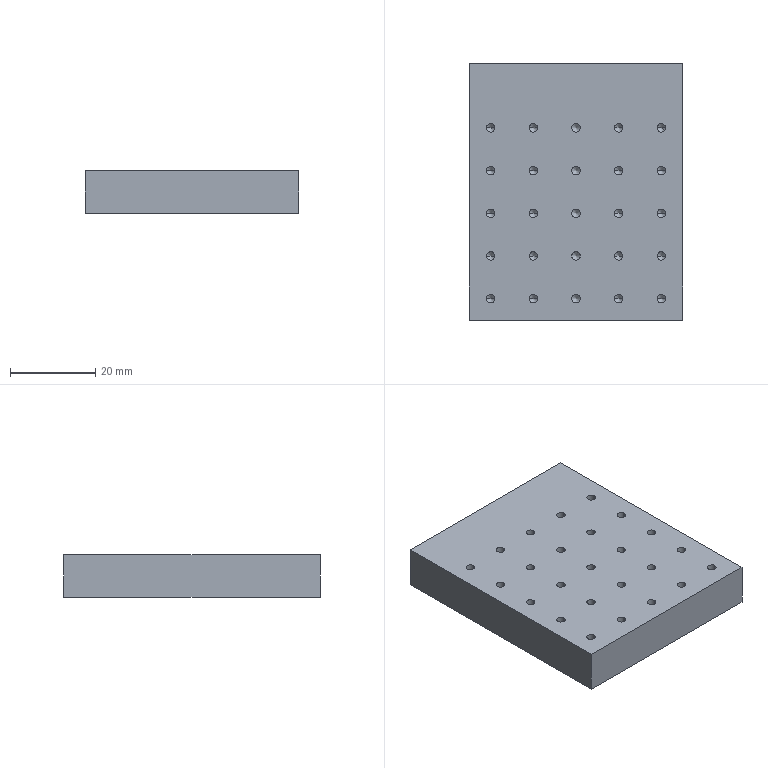Component | SolidWorks | LabelSuctionPlate-1 | 1 solid | 106 faces | box 50 x 60 x 10 mm | volume 29587 mm3 | cylinder 50 | cone 50 | plane 6 | commonest cylinder face diameters 2 x50
build123d program:
from build123d import *

# Parameters (mm, degrees)
SKETCH1_W            = 50
SKETCH1_H            = 60
BOSS_EXTRUDE1_DEPTH  = 10
LPATTERN1_COUNT      = 5
LPATTERN1_PITCH      = 10
LPATTERN1_COUNT_DIR2 = 5
LPATTERN1_PITCH_DIR2 = 10


with BuildPart() as part:
    # Sketch1 → Boss-Extrude1 (new body)
    with BuildSketch(Plane.XY):
        Rectangle(SKETCH1_W, SKETCH1_H)
    extrude(amount=BOSS_EXTRUDE1_DEPTH)

    # Sketch3 → 2.0 _2_ Diameter Hole1 (revolve, cut)
    with BuildSketch(Plane(origin=(20, -25, 10), x_dir=(0, -1, 0), z_dir=(1, 0, 0))):
        Polygon((0, 0), (0, 5.781), (1, 5), (1, 0), align=None)
    f_2_0_2_diameter_hole1 = revolve(axis=Axis((20, -25, 16.35), (0, 0, -1)), mode=Mode.SUBTRACT)

    # LPattern1: 2.0 _2_ Diameter Hole1 5 × 5
    with Locations(*[(-j * LPATTERN1_PITCH_DIR2, i * LPATTERN1_PITCH, 0) for i in range(LPATTERN1_COUNT) for j in range(LPATTERN1_COUNT_DIR2) if (i, j) != (0, 0)]):
        add(f_2_0_2_diameter_hole1, mode=Mode.SUBTRACT)


solid = part.part

# Placed as in the assembly
solid = solid.moved(Location((-45.188, -79.343, 190.72), (0, 0, 0)))